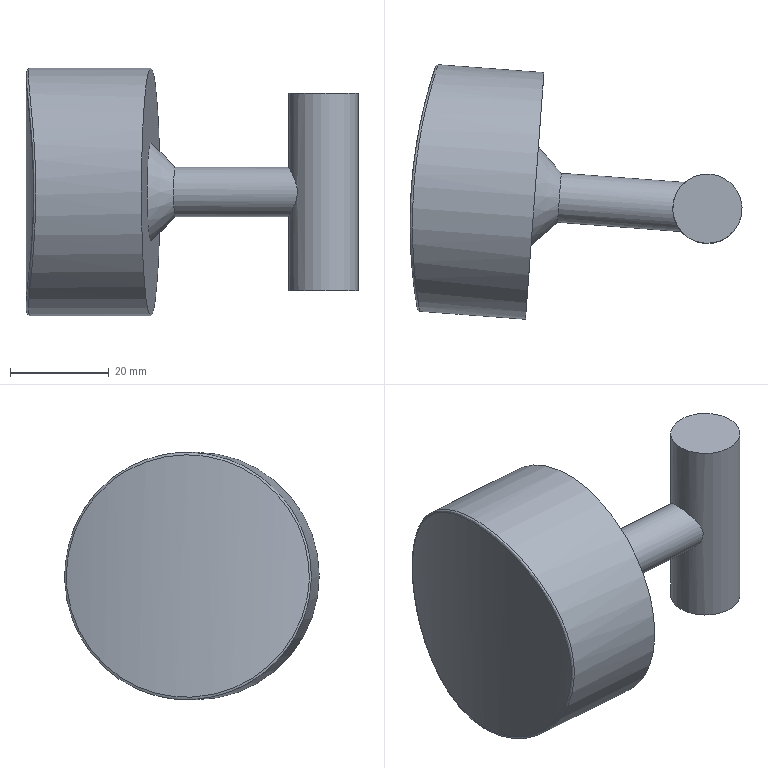Component | NX | PISTON_2 | 1 solid | 9 faces | box 67.11 x 51.46 x 50 mm | volume 56447 mm3 | cylinder 4 | plane 3 | cone 1 | spline 1 | commonest cylinder face diameters 50 x1 14 x1 10 x1 200 x1
STEP:
#1=VALUE_REPRESENTATION_ITEM('',COUNT_MEASURE(0.));
#2=(LENGTH_UNIT()NAMED_UNIT(*)SI_UNIT(.MILLI.,.METRE.));
#3=UNCERTAINTY_MEASURE_WITH_UNIT(LENGTH_MEASURE(0.0508),#2,'','');
#4=(NAMED_UNIT(*)PLANE_ANGLE_UNIT()SI_UNIT($,.RADIAN.));
#5=PLANE_ANGLE_MEASURE_WITH_UNIT(PLANE_ANGLE_MEASURE(0.01745),#4);
#6=DIMENSIONAL_EXPONENTS(0.,0.,0.,0.,0.,0.,0.);
#7=(CONVERSION_BASED_UNIT('',#5)NAMED_UNIT(#6)PLANE_ANGLE_UNIT());
#8=(NAMED_UNIT(*)SI_UNIT($,.STERADIAN.)SOLID_ANGLE_UNIT());
#9=(GEOMETRIC_REPRESENTATION_CONTEXT(3)GLOBAL_UNCERTAINTY_ASSIGNED_CONTEXT((#3))GLOBAL_UNIT_ASSIGNED_CONTEXT((#2,#7,#8))REPRESENTATION_CONTEXT('',''));
#10=REPRESENTATION('',(#1),#9);
#11=VALUE_REPRESENTATION_ITEM('',COUNT_MEASURE(0.));
#12=REPRESENTATION('',(#11),#9);
#13=CARTESIAN_POINT('',(0.,0.,0.));
#14=DIRECTION('',(0.,0.,1.));
#15=DIRECTION('',(1.,0.,0.));
#16=AXIS2_PLACEMENT_3D('',#13,#14,#15);
#17=SHAPE_REPRESENTATION('',(#16),#9);
#18=CARTESIAN_POINT('',(-81.46,14.597,12.5));
#19=VERTEX_POINT('',#18);
#20=CARTESIAN_POINT('',(-81.213,17.904,12.5));
#21=CARTESIAN_POINT('',(-81.708,11.291,12.5));
#22=CARTESIAN_POINT('',(-81.788,8.048,11.85));
#23=CARTESIAN_POINT('',(-81.677,1.931,9.316));
#24=CARTESIAN_POINT('',(-81.489,-0.8324,7.47));
#25=CARTESIAN_POINT('',(-81.037,-5.485,2.857));
#26=CARTESIAN_POINT('',(-80.775,-7.36,0.08605));
#27=CARTESIAN_POINT('',(-80.392,-9.891,-5.93));
#28=CARTESIAN_POINT('',(-80.272,-10.561,-9.231));
#29=CARTESIAN_POINT('',(-80.272,-10.562,-15.765));
#30=CARTESIAN_POINT('',(-80.391,-9.894,-19.062));
#31=CARTESIAN_POINT('',(-80.776,-7.355,-25.097));
#32=CARTESIAN_POINT('',(-81.036,-5.49,-27.854));
#33=CARTESIAN_POINT('',(-81.491,-0.811,-32.489));
#34=CARTESIAN_POINT('',(-81.678,1.947,-34.324));
#35=CARTESIAN_POINT('',(-81.788,8.052,-36.85));
#36=CARTESIAN_POINT('',(-81.704,11.348,-37.501));
#37=CARTESIAN_POINT('',(-81.215,17.869,-37.499));
#38=CARTESIAN_POINT('',(-80.805,21.147,-36.838));
#39=CARTESIAN_POINT('',(-79.797,27.109,-34.337));
#40=CARTESIAN_POINT('',(-79.196,29.842,-32.484));
#41=CARTESIAN_POINT('',(-78.055,34.38,-27.874));
#42=CARTESIAN_POINT('',(-77.521,36.187,-25.133));
#43=CARTESIAN_POINT('',(-76.755,38.664,-19.051));
#44=CARTESIAN_POINT('',(-76.54,39.299,-15.798));
#45=CARTESIAN_POINT('',(-76.539,39.299,-9.206));
#46=CARTESIAN_POINT('',(-76.758,38.655,-5.93));
#47=CARTESIAN_POINT('',(-77.516,36.202,0.09921));
#48=CARTESIAN_POINT('',(-78.056,34.377,2.874));
#49=CARTESIAN_POINT('',(-79.191,29.863,7.465));
#50=CARTESIAN_POINT('',(-79.794,27.125,9.327));
#51=CARTESIAN_POINT('',(-80.802,21.167,11.832));
#52=CARTESIAN_POINT('',(-81.213,17.904,12.5));
#53=CARTESIAN_POINT('',(-81.708,11.291,12.5));
#54=B_SPLINE_CURVE_WITH_KNOTS('',3,(#20,#21,#22,#23,#24,#25,#26,#27,#28,#29,#30,#31,#32,#33,#34,#35,#36,#37,#38,#39,#40,#41,#42,#43,#44,#45,#46,#47,#48,#49,#50,#51,#52,#53),.UNSPECIFIED.,.T.,.F.,(2,2,2,2,2,2,2,2,2,2,2,2,2,2,2,2,2,2,2),(-0.0625,0.,0.0625,0.125,0.1875,0.25,0.3125,0.375,0.4375,0.5,0.5625,0.625,0.6875,0.75,0.8125,0.875,0.9375,1.,1.062),.UNSPECIFIED.);
#55=EDGE_CURVE('',#19,#19,#54,.T.);
#56=ORIENTED_EDGE('',*,*,#55,.T.);
#57=EDGE_LOOP('',(#56));
#58=FACE_BOUND('',#57,.T.);
#59=CARTESIAN_POINT('',(-57.029,12.769,12.5));
#60=VERTEX_POINT('',#59);
#61=CARTESIAN_POINT('',(-57.029,12.769,-12.5));
#62=DIRECTION('',(-0.9972,0.07464,0.));
#63=DIRECTION('',(0.,0.,1.));
#64=AXIS2_PLACEMENT_3D('',#61,#62,#63);
#65=CIRCLE('',#64,25.);
#66=EDGE_CURVE('',#60,#60,#65,.T.);
#67=ORIENTED_EDGE('',*,*,#66,.T.);
#68=EDGE_LOOP('',(#67));
#69=FACE_BOUND('',#68,.T.);
#70=CARTESIAN_POINT('',(-57.029,12.769,-12.5));
#71=DIRECTION('',(-0.9972,0.07464,0.));
#72=DIRECTION('',(0.,0.,1.));
#73=AXIS2_PLACEMENT_3D('',#70,#71,#72);
#74=CYLINDRICAL_SURFACE('',#73,25.);
#75=ADVANCED_FACE('',(#58,#69),#74,.T.);
#76=CARTESIAN_POINT('',(-21.604,17.137,-32.5));
#77=VERTEX_POINT('',#76);
#78=CARTESIAN_POINT('',(-22.126,10.156,-32.5));
#79=DIRECTION('',(0.,0.,-1.));
#80=DIRECTION('',(0.07464,0.9972,0.));
#81=AXIS2_PLACEMENT_3D('',#78,#79,#80);
#82=CIRCLE('',#81,7.);
#83=EDGE_CURVE('',#77,#77,#82,.T.);
#84=ORIENTED_EDGE('',*,*,#83,.F.);
#85=EDGE_LOOP('',(#84));
#86=FACE_BOUND('',#85,.T.);
#87=CARTESIAN_POINT('',(-21.604,17.137,7.5));
#88=VERTEX_POINT('',#87);
#89=CARTESIAN_POINT('',(-22.126,10.156,7.5));
#90=DIRECTION('',(0.,0.,-1.));
#91=DIRECTION('',(0.07464,0.9972,0.));
#92=AXIS2_PLACEMENT_3D('',#89,#90,#91);
#93=CIRCLE('',#92,7.);
#94=EDGE_CURVE('',#88,#88,#93,.T.);
#95=ORIENTED_EDGE('',*,*,#94,.T.);
#96=EDGE_LOOP('',(#95));
#97=FACE_BOUND('',#96,.T.);
#98=CARTESIAN_POINT('',(-29.107,10.679,-7.5));
#99=VERTEX_POINT('',#98);
#100=CARTESIAN_POINT('',(-29.004,12.053,-7.5));
#101=CARTESIAN_POINT('',(-29.21,9.304,-7.5));
#102=CARTESIAN_POINT('',(-28.862,7.99,-8.085));
#103=CARTESIAN_POINT('',(-27.954,6.143,-9.873));
#104=CARTESIAN_POINT('',(-27.386,5.537,-11.136));
#105=CARTESIAN_POINT('',(-27.384,5.535,-13.858));
#106=CARTESIAN_POINT('',(-27.948,6.135,-15.115));
#107=CARTESIAN_POINT('',(-28.86,7.984,-16.913));
#108=CARTESIAN_POINT('',(-29.207,9.31,-17.497));
#109=CARTESIAN_POINT('',(-29.009,12.023,-17.503));
#110=CARTESIAN_POINT('',(-28.468,13.296,-16.92));
#111=CARTESIAN_POINT('',(-27.29,14.994,-15.126));
#112=CARTESIAN_POINT('',(-26.639,15.507,-13.876));
#113=CARTESIAN_POINT('',(-26.638,15.508,-11.128));
#114=CARTESIAN_POINT('',(-27.292,14.991,-9.872));
#115=CARTESIAN_POINT('',(-28.465,13.3,-8.084));
#116=CARTESIAN_POINT('',(-29.004,12.053,-7.5));
#117=CARTESIAN_POINT('',(-29.21,9.304,-7.5));
#118=B_SPLINE_CURVE_WITH_KNOTS('',3,(#100,#101,#102,#103,#104,#105,#106,#107,#108,#109,#110,#111,#112,#113,#114,#115,#116,#117),.UNSPECIFIED.,.T.,.F.,(2,2,2,2,2,2,2,2,2,2,2),(-0.125,0.,0.125,0.25,0.375,0.5,0.625,0.75,0.875,1.,1.125),.UNSPECIFIED.);
#119=EDGE_CURVE('',#99,#99,#118,.T.);
#120=ORIENTED_EDGE('',*,*,#119,.T.);
#121=EDGE_LOOP('',(#120));
#122=FACE_BOUND('',#121,.T.);
#123=CARTESIAN_POINT('',(-22.126,10.156,7.5));
#124=DIRECTION('',(0.,0.,-1.));
#125=DIRECTION('',(-0.9972,0.07464,0.));
#126=AXIS2_PLACEMENT_3D('',#123,#124,#125);
#127=CYLINDRICAL_SURFACE('',#126,7.);
#128=ADVANCED_FACE('',(#86,#97,#122),#127,.T.);
#129=ORIENTED_EDGE('',*,*,#94,.F.);
#130=EDGE_LOOP('',(#129));
#131=FACE_OUTER_BOUND('',#130,.T.);
#132=CARTESIAN_POINT('',(-22.126,10.156,7.5));
#133=DIRECTION('',(0.,0.,-1.));
#134=DIRECTION('',(-0.9972,0.07464,0.));
#135=AXIS2_PLACEMENT_3D('',#132,#133,#134);
#136=PLANE('',#135);
#137=ADVANCED_FACE('',(#131),#136,.F.);
#138=ORIENTED_EDGE('',*,*,#83,.T.);
#139=EDGE_LOOP('',(#138));
#140=FACE_OUTER_BOUND('',#139,.T.);
#141=CARTESIAN_POINT('',(-22.126,10.156,-32.5));
#142=DIRECTION('',(0.,0.,-1.));
#143=DIRECTION('',(-0.9972,0.07464,0.));
#144=AXIS2_PLACEMENT_3D('',#141,#142,#143);
#145=PLANE('',#144);
#146=ADVANCED_FACE('',(#140),#145,.T.);
#147=CARTESIAN_POINT('',(-52.043,12.395,-17.5));
#148=VERTEX_POINT('',#147);
#149=CARTESIAN_POINT('',(-52.043,12.395,-12.5));
#150=DIRECTION('',(0.9972,-0.07464,0.));
#151=DIRECTION('',(0.,0.,-1.));
#152=AXIS2_PLACEMENT_3D('',#149,#150,#151);
#153=CIRCLE('',#152,5.);
#154=EDGE_CURVE('',#148,#148,#153,.T.);
#155=ORIENTED_EDGE('',*,*,#154,.T.);
#156=EDGE_LOOP('',(#155));
#157=FACE_BOUND('',#156,.T.);
#158=ORIENTED_EDGE('',*,*,#119,.F.);
#159=EDGE_LOOP('',(#158));
#160=FACE_BOUND('',#159,.T.);
#161=CARTESIAN_POINT('',(-57.029,12.769,-12.5));
#162=DIRECTION('',(0.9972,-0.07464,0.));
#163=DIRECTION('',(0.,0.,-1.));
#164=AXIS2_PLACEMENT_3D('',#161,#162,#163);
#165=CYLINDRICAL_SURFACE('',#164,5.);
#166=ADVANCED_FACE('',(#157,#160),#165,.T.);
#167=CARTESIAN_POINT('',(-57.029,12.769,-22.5));
#168=VERTEX_POINT('',#167);
#169=CARTESIAN_POINT('',(-57.029,12.769,-12.5));
#170=DIRECTION('',(-0.9972,0.07464,0.));
#171=DIRECTION('',(0.,0.,-1.));
#172=AXIS2_PLACEMENT_3D('',#169,#170,#171);
#173=CIRCLE('',#172,10.);
#174=EDGE_CURVE('',#168,#168,#173,.T.);
#175=ORIENTED_EDGE('',*,*,#174,.T.);
#176=EDGE_LOOP('',(#175));
#177=FACE_BOUND('',#176,.T.);
#178=ORIENTED_EDGE('',*,*,#66,.F.);
#179=EDGE_LOOP('',(#178));
#180=FACE_BOUND('',#179,.T.);
#181=CARTESIAN_POINT('',(-57.029,12.769,-12.5));
#182=DIRECTION('',(0.9972,-0.07464,0.));
#183=DIRECTION('',(0.,0.,-1.));
#184=AXIS2_PLACEMENT_3D('',#181,#182,#183);
#185=PLANE('',#184);
#186=ADVANCED_FACE('',(#177,#180),#185,.T.);
#187=ORIENTED_EDGE('',*,*,#154,.F.);
#188=EDGE_LOOP('',(#187));
#189=FACE_BOUND('',#188,.T.);
#190=ORIENTED_EDGE('',*,*,#174,.F.);
#191=EDGE_LOOP('',(#190));
#192=FACE_BOUND('',#191,.T.);
#193=CARTESIAN_POINT('',(-57.029,12.769,-12.5));
#194=DIRECTION('',(-0.9972,0.07464,0.));
#195=DIRECTION('',(0.,0.,1.));
#196=AXIS2_PLACEMENT_3D('',#193,#194,#195);
#197=CONICAL_SURFACE('',#196,10.,45.);
#198=ADVANCED_FACE('',(#189,#192),#197,.T.);
#199=CARTESIAN_POINT('',(-81.959,14.635,12.));
#200=VERTEX_POINT('',#199);
#201=CARTESIAN_POINT('',(-82.202,11.386,12.));
#202=CARTESIAN_POINT('',(-81.716,17.884,12.));
#203=CARTESIAN_POINT('',(-81.309,21.089,11.349));
#204=CARTESIAN_POINT('',(-80.307,26.951,8.903));
#205=CARTESIAN_POINT('',(-79.706,29.646,7.083));
#206=CARTESIAN_POINT('',(-78.572,34.096,2.59));
#207=CARTESIAN_POINT('',(-78.031,35.897,-0.1297));
#208=CARTESIAN_POINT('',(-77.271,38.321,-6.046));
#209=CARTESIAN_POINT('',(-77.051,38.96,-9.264));
#210=CARTESIAN_POINT('',(-77.051,38.959,-15.742));
#211=CARTESIAN_POINT('',(-77.268,38.329,-18.939));
#212=CARTESIAN_POINT('',(-78.037,35.881,-24.907));
#213=CARTESIAN_POINT('',(-78.572,34.097,-27.592));
#214=CARTESIAN_POINT('',(-79.712,29.623,-32.103));
#215=CARTESIAN_POINT('',(-80.311,26.933,-33.913));
#216=CARTESIAN_POINT('',(-81.312,21.07,-36.354));
#217=CARTESIAN_POINT('',(-81.718,17.848,-36.999));
#218=CARTESIAN_POINT('',(-82.198,11.44,-37.001));
#219=CARTESIAN_POINT('',(-82.278,8.201,-36.366));
#220=CARTESIAN_POINT('',(-82.159,2.197,-33.9));
#221=CARTESIAN_POINT('',(-81.969,-0.5194,-32.107));
#222=CARTESIAN_POINT('',(-81.505,-5.134,-27.571));
#223=CARTESIAN_POINT('',(-81.24,-6.977,-24.869));
#224=CARTESIAN_POINT('',(-80.849,-9.488,-18.947));
#225=CARTESIAN_POINT('',(-80.727,-10.15,-15.707));
#226=CARTESIAN_POINT('',(-80.727,-10.149,-9.287));
#227=CARTESIAN_POINT('',(-80.849,-9.485,-6.044));
#228=CARTESIAN_POINT('',(-81.24,-6.981,-0.1406));
#229=CARTESIAN_POINT('',(-81.506,-5.128,2.575));
#230=CARTESIAN_POINT('',(-81.967,-0.5396,7.089));
#231=CARTESIAN_POINT('',(-82.159,2.181,8.892));
#232=CARTESIAN_POINT('',(-82.278,8.199,11.366));
#233=CARTESIAN_POINT('',(-82.202,11.386,12.));
#234=CARTESIAN_POINT('',(-81.716,17.884,12.));
#235=B_SPLINE_CURVE_WITH_KNOTS('',3,(#201,#202,#203,#204,#205,#206,#207,#208,#209,#210,#211,#212,#213,#214,#215,#216,#217,#218,#219,#220,#221,#222,#223,#224,#225,#226,#227,#228,#229,#230,#231,#232,#233,#234),.UNSPECIFIED.,.T.,.F.,(2,2,2,2,2,2,2,2,2,2,2,2,2,2,2,2,2,2,2),(-0.0625,0.,0.0625,0.125,0.1875,0.25,0.3125,0.375,0.4375,0.5,0.5625,0.625,0.6875,0.75,0.8125,0.875,0.9375,1.,1.062),.UNSPECIFIED.);
#236=EDGE_CURVE('',#200,#200,#235,.T.);
#237=ORIENTED_EDGE('',*,*,#236,.T.);
#238=EDGE_LOOP('',(#237));
#239=FACE_OUTER_BOUND('',#238,.T.);
#240=CARTESIAN_POINT('',(17.762,7.17,22.5));
#241=DIRECTION('',(0.,0.,-1.));
#242=DIRECTION('',(-0.9972,0.07464,0.));
#243=AXIS2_PLACEMENT_3D('',#240,#241,#242);
#244=CYLINDRICAL_SURFACE('',#243,100.);
#245=ADVANCED_FACE('',(#239),#244,.T.);
#246=ORIENTED_EDGE('',*,*,#236,.F.);
#247=EDGE_LOOP('',(#246));
#248=FACE_BOUND('',#247,.T.);
#249=ORIENTED_EDGE('',*,*,#55,.F.);
#250=EDGE_LOOP('',(#249));
#251=FACE_BOUND('',#250,.T.);
#252=CARTESIAN_POINT('',(-81.228,21.349,11.061));
#253=CARTESIAN_POINT('',(-81.209,21.482,11.534));
#254=CARTESIAN_POINT('',(-80.723,21.415,11.542));
#255=CARTESIAN_POINT('',(-81.451,19.794,11.506));
#256=CARTESIAN_POINT('',(-81.439,19.891,11.993));
#257=CARTESIAN_POINT('',(-80.947,19.836,11.996));
#258=CARTESIAN_POINT('',(-81.639,18.217,11.79));
#259=CARTESIAN_POINT('',(-81.632,18.288,12.284));
#260=CARTESIAN_POINT('',(-81.136,18.235,12.286));
#261=CARTESIAN_POINT('',(-81.942,15.023,12.049));
#262=CARTESIAN_POINT('',(-81.942,15.029,12.551));
#263=CARTESIAN_POINT('',(-81.443,14.991,12.55));
#264=CARTESIAN_POINT('',(-82.058,13.386,12.021));
#265=CARTESIAN_POINT('',(-82.06,13.363,12.522));
#266=CARTESIAN_POINT('',(-81.56,13.329,12.522));
#267=CARTESIAN_POINT('',(-82.206,10.171,11.647));
#268=CARTESIAN_POINT('',(-82.209,10.084,12.136));
#269=CARTESIAN_POINT('',(-81.713,10.066,12.14));
#270=CARTESIAN_POINT('',(-82.24,8.598,11.305));
#271=CARTESIAN_POINT('',(-82.242,8.484,11.787));
#272=CARTESIAN_POINT('',(-81.749,8.469,11.791));
#273=CARTESIAN_POINT('',(-82.236,5.52,10.318));
#274=CARTESIAN_POINT('',(-82.234,5.348,10.771));
#275=CARTESIAN_POINT('',(-81.75,5.343,10.784));
#276=CARTESIAN_POINT('',(-82.198,4.012,9.666));
#277=CARTESIAN_POINT('',(-82.192,3.816,10.104));
#278=CARTESIAN_POINT('',(-81.714,3.813,10.118));
#279=CARTESIAN_POINT('',(-82.005,-0.2136,7.331));
#280=CARTESIAN_POINT('',(-81.988,-0.4519,7.723));
#281=CARTESIAN_POINT('',(-81.528,-0.4766,7.736));
#282=CARTESIAN_POINT('',(-81.766,-2.742,5.209));
#283=CARTESIAN_POINT('',(-81.739,-3.023,5.565));
#284=CARTESIAN_POINT('',(-81.295,-3.043,5.57));
#285=CARTESIAN_POINT('',(-81.404,-5.755,1.469));
#286=CARTESIAN_POINT('',(-81.361,-6.092,1.721));
#287=CARTESIAN_POINT('',(-80.939,-6.102,1.754));
#288=CARTESIAN_POINT('',(-81.281,-6.648,0.1094));
#289=CARTESIAN_POINT('',(-81.233,-6.997,0.3348));
#290=CARTESIAN_POINT('',(-80.818,-7.008,0.3667));
#291=CARTESIAN_POINT('',(-81.062,-8.142,-2.748));
#292=CARTESIAN_POINT('',(-81.006,-8.504,-2.575));
#293=CARTESIAN_POINT('',(-80.602,-8.524,-2.549));
#294=CARTESIAN_POINT('',(-80.965,-8.739,-4.232));
#295=CARTESIAN_POINT('',(-80.906,-9.109,-4.088));
#296=CARTESIAN_POINT('',(-80.507,-9.13,-4.063));
#297=CARTESIAN_POINT('',(-80.817,-9.637,-7.311));
#298=CARTESIAN_POINT('',(-80.752,-10.014,-7.22));
#299=CARTESIAN_POINT('',(-80.36,-10.041,-7.205));
#300=CARTESIAN_POINT('',(-80.764,-9.936,-8.922));
#301=CARTESIAN_POINT('',(-80.698,-10.317,-8.862));
#302=CARTESIAN_POINT('',(-80.309,-10.344,-8.849));
#303=CARTESIAN_POINT('',(-80.718,-10.2,-12.122));
#304=CARTESIAN_POINT('',(-80.65,-10.583,-12.114));
#305=CARTESIAN_POINT('',(-80.263,-10.613,-12.114));
#306=CARTESIAN_POINT('',(-80.723,-10.173,-13.724));
#307=CARTESIAN_POINT('',(-80.655,-10.556,-13.746));
#308=CARTESIAN_POINT('',(-80.268,-10.585,-13.749));
#309=CARTESIAN_POINT('',(-80.822,-9.602,-18.535));
#310=CARTESIAN_POINT('',(-80.758,-9.979,-18.644));
#311=CARTESIAN_POINT('',(-80.366,-10.006,-18.658));
#312=CARTESIAN_POINT('',(-81.004,-8.576,-21.636));
#313=CARTESIAN_POINT('',(-80.947,-8.929,-21.821));
#314=CARTESIAN_POINT('',(-80.545,-8.965,-21.822));
#315=CARTESIAN_POINT('',(-81.346,-6.179,-25.85));
#316=CARTESIAN_POINT('',(-81.3,-6.522,-26.09));
#317=CARTESIAN_POINT('',(-80.882,-6.531,-26.123));
#318=CARTESIAN_POINT('',(-81.469,-5.253,-27.157));
#319=CARTESIAN_POINT('',(-81.428,-5.583,-27.424));
#320=CARTESIAN_POINT('',(-81.003,-5.591,-27.457));
#321=CARTESIAN_POINT('',(-81.709,-3.154,-29.585));
#322=CARTESIAN_POINT('',(-81.678,-3.46,-29.903));
#323=CARTESIAN_POINT('',(-81.239,-3.461,-29.934));
#324=CARTESIAN_POINT('',(-81.828,-1.968,-30.714));
#325=CARTESIAN_POINT('',(-81.801,-2.256,-31.055));
#326=CARTESIAN_POINT('',(-81.355,-2.257,-31.085));
#327=CARTESIAN_POINT('',(-82.028,0.5674,-32.695));
#328=CARTESIAN_POINT('',(-82.012,0.3154,-33.084));
#329=CARTESIAN_POINT('',(-81.55,0.3162,-33.107));
#330=CARTESIAN_POINT('',(-82.111,1.921,-33.557));
#331=CARTESIAN_POINT('',(-82.099,1.69,-33.965));
#332=CARTESIAN_POINT('',(-81.63,1.691,-33.987));
#333=CARTESIAN_POINT('',(-82.22,4.805,-35.024));
#334=CARTESIAN_POINT('',(-82.217,4.623,-35.471));
#335=CARTESIAN_POINT('',(-81.735,4.618,-35.483));
#336=CARTESIAN_POINT('',(-82.247,6.332,-35.621));
#337=CARTESIAN_POINT('',(-82.246,6.175,-36.083));
#338=CARTESIAN_POINT('',(-81.759,6.168,-36.093));
#339=CARTESIAN_POINT('',(-82.224,9.441,-36.501));
#340=CARTESIAN_POINT('',(-82.227,9.343,-36.988));
#341=CARTESIAN_POINT('',(-81.732,9.324,-36.991));
#342=CARTESIAN_POINT('',(-82.176,11.055,-36.792));
#343=CARTESIAN_POINT('',(-82.179,10.985,-37.286));
#344=CARTESIAN_POINT('',(-81.681,10.963,-37.288));
#345=CARTESIAN_POINT('',(-81.998,14.28,-37.05));
#346=CARTESIAN_POINT('',(-81.999,14.275,-37.552));
#347=CARTESIAN_POINT('',(-81.5,14.238,-37.551));
#348=CARTESIAN_POINT('',(-81.87,15.885,-37.021));
#349=CARTESIAN_POINT('',(-81.869,15.908,-37.522));
#350=CARTESIAN_POINT('',(-81.37,15.867,-37.521));
#351=CARTESIAN_POINT('',(-81.539,19.079,-36.648));
#352=CARTESIAN_POINT('',(-81.529,19.166,-37.137));
#353=CARTESIAN_POINT('',(-81.036,19.11,-37.141));
#354=CARTESIAN_POINT('',(-81.334,20.674,-36.298));
#355=CARTESIAN_POINT('',(-81.319,20.787,-36.779));
#356=CARTESIAN_POINT('',(-80.829,20.729,-36.784));
#357=CARTESIAN_POINT('',(-80.873,23.707,-35.311));
#358=CARTESIAN_POINT('',(-80.845,23.876,-35.764));
#359=CARTESIAN_POINT('',(-80.366,23.809,-35.776));
#360=CARTESIAN_POINT('',(-80.616,25.164,-34.672));
#361=CARTESIAN_POINT('',(-80.581,25.357,-35.11));
#362=CARTESIAN_POINT('',(-80.108,25.289,-35.125));
#363=CARTESIAN_POINT('',(-80.064,27.96,-33.099));
#364=CARTESIAN_POINT('',(-80.013,28.197,-33.496));
#365=CARTESIAN_POINT('',(-79.554,28.128,-33.519));
#366=CARTESIAN_POINT('',(-79.775,29.263,-32.182));
#367=CARTESIAN_POINT('',(-79.717,29.52,-32.558));
#368=CARTESIAN_POINT('',(-79.265,29.451,-32.583));
#369=CARTESIAN_POINT('',(-79.201,31.661,-30.118));
#370=CARTESIAN_POINT('',(-79.128,31.951,-30.447));
#371=CARTESIAN_POINT('',(-78.69,31.887,-30.478));
#372=CARTESIAN_POINT('',(-78.911,32.771,-28.956));
#373=CARTESIAN_POINT('',(-78.83,33.076,-29.26));
#374=CARTESIAN_POINT('',(-78.4,33.014,-29.291));
#375=CARTESIAN_POINT('',(-78.37,34.733,-26.443));
#376=CARTESIAN_POINT('',(-78.276,35.059,-26.696));
#377=CARTESIAN_POINT('',(-77.858,35.007,-26.728));
#378=CARTESIAN_POINT('',(-78.12,35.582,-25.105));
#379=CARTESIAN_POINT('',(-78.02,35.919,-25.33));
#380=CARTESIAN_POINT('',(-77.609,35.868,-25.362));
#381=CARTESIAN_POINT('',(-77.682,37.019,-22.263));
#382=CARTESIAN_POINT('',(-77.573,37.369,-22.435));
#383=CARTESIAN_POINT('',(-77.171,37.328,-22.462));
#384=CARTESIAN_POINT('',(-77.494,37.609,-20.744));
#385=CARTESIAN_POINT('',(-77.38,37.966,-20.887));
#386=CARTESIAN_POINT('',(-76.983,37.927,-20.912));
#387=CARTESIAN_POINT('',(-77.214,38.471,-17.664));
#388=CARTESIAN_POINT('',(-77.094,38.835,-17.754));
#389=CARTESIAN_POINT('',(-76.703,38.803,-17.769));
#390=CARTESIAN_POINT('',(-77.12,38.752,-16.09));
#391=CARTESIAN_POINT('',(-76.998,39.119,-16.151));
#392=CARTESIAN_POINT('',(-76.609,39.089,-16.163));
#393=CARTESIAN_POINT('',(-77.034,39.009,-12.872));
#394=CARTESIAN_POINT('',(-76.91,39.378,-12.88));
#395=CARTESIAN_POINT('',(-76.523,39.349,-12.88));
#396=CARTESIAN_POINT('',(-77.044,38.979,-11.244));
#397=CARTESIAN_POINT('',(-76.921,39.348,-11.221));
#398=CARTESIAN_POINT('',(-76.533,39.319,-11.218));
#399=CARTESIAN_POINT('',(-77.227,38.43,-6.473));
#400=CARTESIAN_POINT('',(-77.108,38.794,-6.364));
#401=CARTESIAN_POINT('',(-76.716,38.762,-6.35));
#402=CARTESIAN_POINT('',(-77.563,37.432,-3.341));
#403=CARTESIAN_POINT('',(-77.455,37.773,-3.156));
#404=CARTESIAN_POINT('',(-77.051,37.748,-3.154));
#405=CARTESIAN_POINT('',(-78.253,35.131,0.8399));
#406=CARTESIAN_POINT('',(-78.156,35.463,1.08));
#407=CARTESIAN_POINT('',(-77.742,35.41,1.112));
#408=CARTESIAN_POINT('',(-78.517,34.215,2.175));
#409=CARTESIAN_POINT('',(-78.427,34.536,2.441));
#410=CARTESIAN_POINT('',(-78.006,34.48,2.474));
#411=CARTESIAN_POINT('',(-79.068,32.171,4.603));
#412=CARTESIAN_POINT('',(-78.992,32.468,4.921));
#413=CARTESIAN_POINT('',(-78.557,32.404,4.952));
#414=CARTESIAN_POINT('',(-79.356,31.04,5.708));
#415=CARTESIAN_POINT('',(-79.287,31.321,6.049));
#416=CARTESIAN_POINT('',(-78.845,31.256,6.079));
#417=CARTESIAN_POINT('',(-79.933,28.553,7.697));
#418=CARTESIAN_POINT('',(-79.88,28.8,8.086));
#419=CARTESIAN_POINT('',(-79.424,28.731,8.109));
#420=CARTESIAN_POINT('',(-80.222,27.202,8.573));
#421=CARTESIAN_POINT('',(-80.176,27.428,8.981));
#422=CARTESIAN_POINT('',(-79.713,27.358,9.003));
#423=CARTESIAN_POINT('',(-80.756,24.384,10.027));
#424=CARTESIAN_POINT('',(-80.725,24.563,10.475));
#425=CARTESIAN_POINT('',(-80.248,24.496,10.487));
#426=CARTESIAN_POINT('',(-81.005,22.904,10.617));
#427=CARTESIAN_POINT('',(-80.981,23.06,11.078));
#428=CARTESIAN_POINT('',(-80.499,22.994,11.089));
#429=CARTESIAN_POINT('',(-81.228,21.349,11.061));
#430=CARTESIAN_POINT('',(-81.209,21.482,11.534));
#431=CARTESIAN_POINT('',(-80.723,21.415,11.542));
#432=(BOUNDED_SURFACE()B_SPLINE_SURFACE(3,2,((#252,#253,#254),(#255,#256,#257),(#258,#259,#260),(#261,#262,#263),(#264,#265,#266),(#267,#268,#269),(#270,#271,#272),(#273,#274,#275),(#276,#277,#278),(#279,#280,#281),(#282,#283,#284),(#285,#286,#287),(#288,#289,#290),(#291,#292,#293),(#294,#295,#296),(#297,#298,#299),(#300,#301,#302),(#303,#304,#305),(#306,#307,#308),(#309,#310,#311),(#312,#313,#314),(#315,#316,#317),(#318,#319,#320),(#321,#322,#323),(#324,#325,#326),(#327,#328,#329),(#330,#331,#332),(#333,#334,#335),(#336,#337,#338),(#339,#340,#341),(#342,#343,#344),(#345,#346,#347),(#348,#349,#350),(#351,#352,#353),(#354,#355,#356),(#357,#358,#359),(#360,#361,#362),(#363,#364,#365),(#366,#367,#368),(#369,#370,#371),(#372,#373,#374),(#375,#376,#377),(#378,#379,#380),(#381,#382,#383),(#384,#385,#386),(#387,#388,#389),(#390,#391,#392),(#393,#394,#395),(#396,#397,#398),(#399,#400,#401),(#402,#403,#404),(#405,#406,#407),(#408,#409,#410),(#411,#412,#413),(#414,#415,#416),(#417,#418,#419),(#420,#421,#422),(#423,#424,#425),(#426,#427,#428),(#429,#430,#431)),.UNSPECIFIED.,.T.,.F.,.F.)B_SPLINE_SURFACE_WITH_KNOTS((1,3,2,2,2,2,2,2,2,2,2,2,2,2,2,2,2,2,2,2,2,2,2,2,2,2,2,2,2,2,3,1),(3,3),(-0.03125,0.,0.03125,0.0625,0.09375,0.125,0.1875,0.2188,0.25,0.2812,0.3125,0.375,0.4062,0.4375,0.4688,0.5,0.5312,0.5625,0.5938,0.625,0.6562,0.6875,0.7188,0.75,0.7812,0.8125,0.875,0.9062,0.9375,0.9688,1.,1.031),(0.,1.),.UNSPECIFIED.)GEOMETRIC_REPRESENTATION_ITEM()RATIONAL_B_SPLINE_SURFACE(((1.,0.7136,1.),(1.,0.7106,1.),(1.,0.7086,1.),(1.,0.7068,1.),(1.,0.707,1.),(1.,0.7096,1.),(1.,0.712,1.),(1.,0.7186,1.),(1.,0.7228,1.),(1.,0.7369,1.),(1.,0.7484,1.),(1.,0.7638,1.),(1.,0.7687,1.),(1.,0.7772,1.),(1.,0.7808,1.),(1.,0.7862,1.),(1.,0.788,1.),(1.,0.7897,1.),(1.,0.7895,1.),(1.,0.786,1.),(1.,0.7795,1.),(1.,0.7661,1.),(1.,0.7612,1.),(1.,0.7507,1.),(1.,0.7452,1.),(1.,0.7346,1.),(1.,0.7296,1.),(1.,0.7205,1.),(1.,0.7166,1.),(1.,0.7106,1.),(1.,0.7086,1.),(1.,0.7068,1.),(1.,0.707,1.),(1.,0.7096,1.),(1.,0.712,1.),(1.,0.7186,1.),(1.,0.7228,1.),(1.,0.7323,1.),(1.,0.7375,1.),(1.,0.7481,1.),(1.,0.7536,1.),(1.,0.7639,1.),(1.,0.7687,1.),(1.,0.7772,1.),(1.,0.7808,1.),(1.,0.7862,1.),(1.,0.788,1.),(1.,0.7897,1.),(1.,0.7895,1.),(1.,0.786,1.),(1.,0.7795,1.),(1.,0.7662,1.),(1.,0.7611,1.),(1.,0.7506,1.),(1.,0.7452,1.),(1.,0.7346,1.),(1.,0.7295,1.),(1.,0.7205,1.),(1.,0.7166,1.),(1.,0.7136,1.)))REPRESENTATION_ITEM('')SURFACE());
#433=ADVANCED_FACE('',(#248,#251),#432,.T.);
#434=CLOSED_SHELL('',(#75,#128,#137,#146,#166,#186,#198,#245,#433));
#435=MANIFOLD_SOLID_BREP('',#434);
#436=ADVANCED_BREP_SHAPE_REPRESENTATION('',(#435),#9);
#437=SHAPE_REPRESENTATION_RELATIONSHIP('','',#17,#436);
#438=PRESENTATION_LAYER_ASSIGNMENT('','',(#435));
#439=COLOUR_RGB('',1.,0.6,0.);
#440=FILL_AREA_STYLE_COLOUR('',#439);
#441=FILL_AREA_STYLE('',(#440));
#442=SURFACE_STYLE_FILL_AREA(#441);
#443=SURFACE_SIDE_STYLE('',(#442));
#444=SURFACE_STYLE_USAGE(.BOTH.,#443);
#445=PRESENTATION_STYLE_ASSIGNMENT((#444));
#446=STYLED_ITEM('',(#445),#435);
#447=MECHANICAL_DESIGN_GEOMETRIC_PRESENTATION_REPRESENTATION('',(#446),#9);